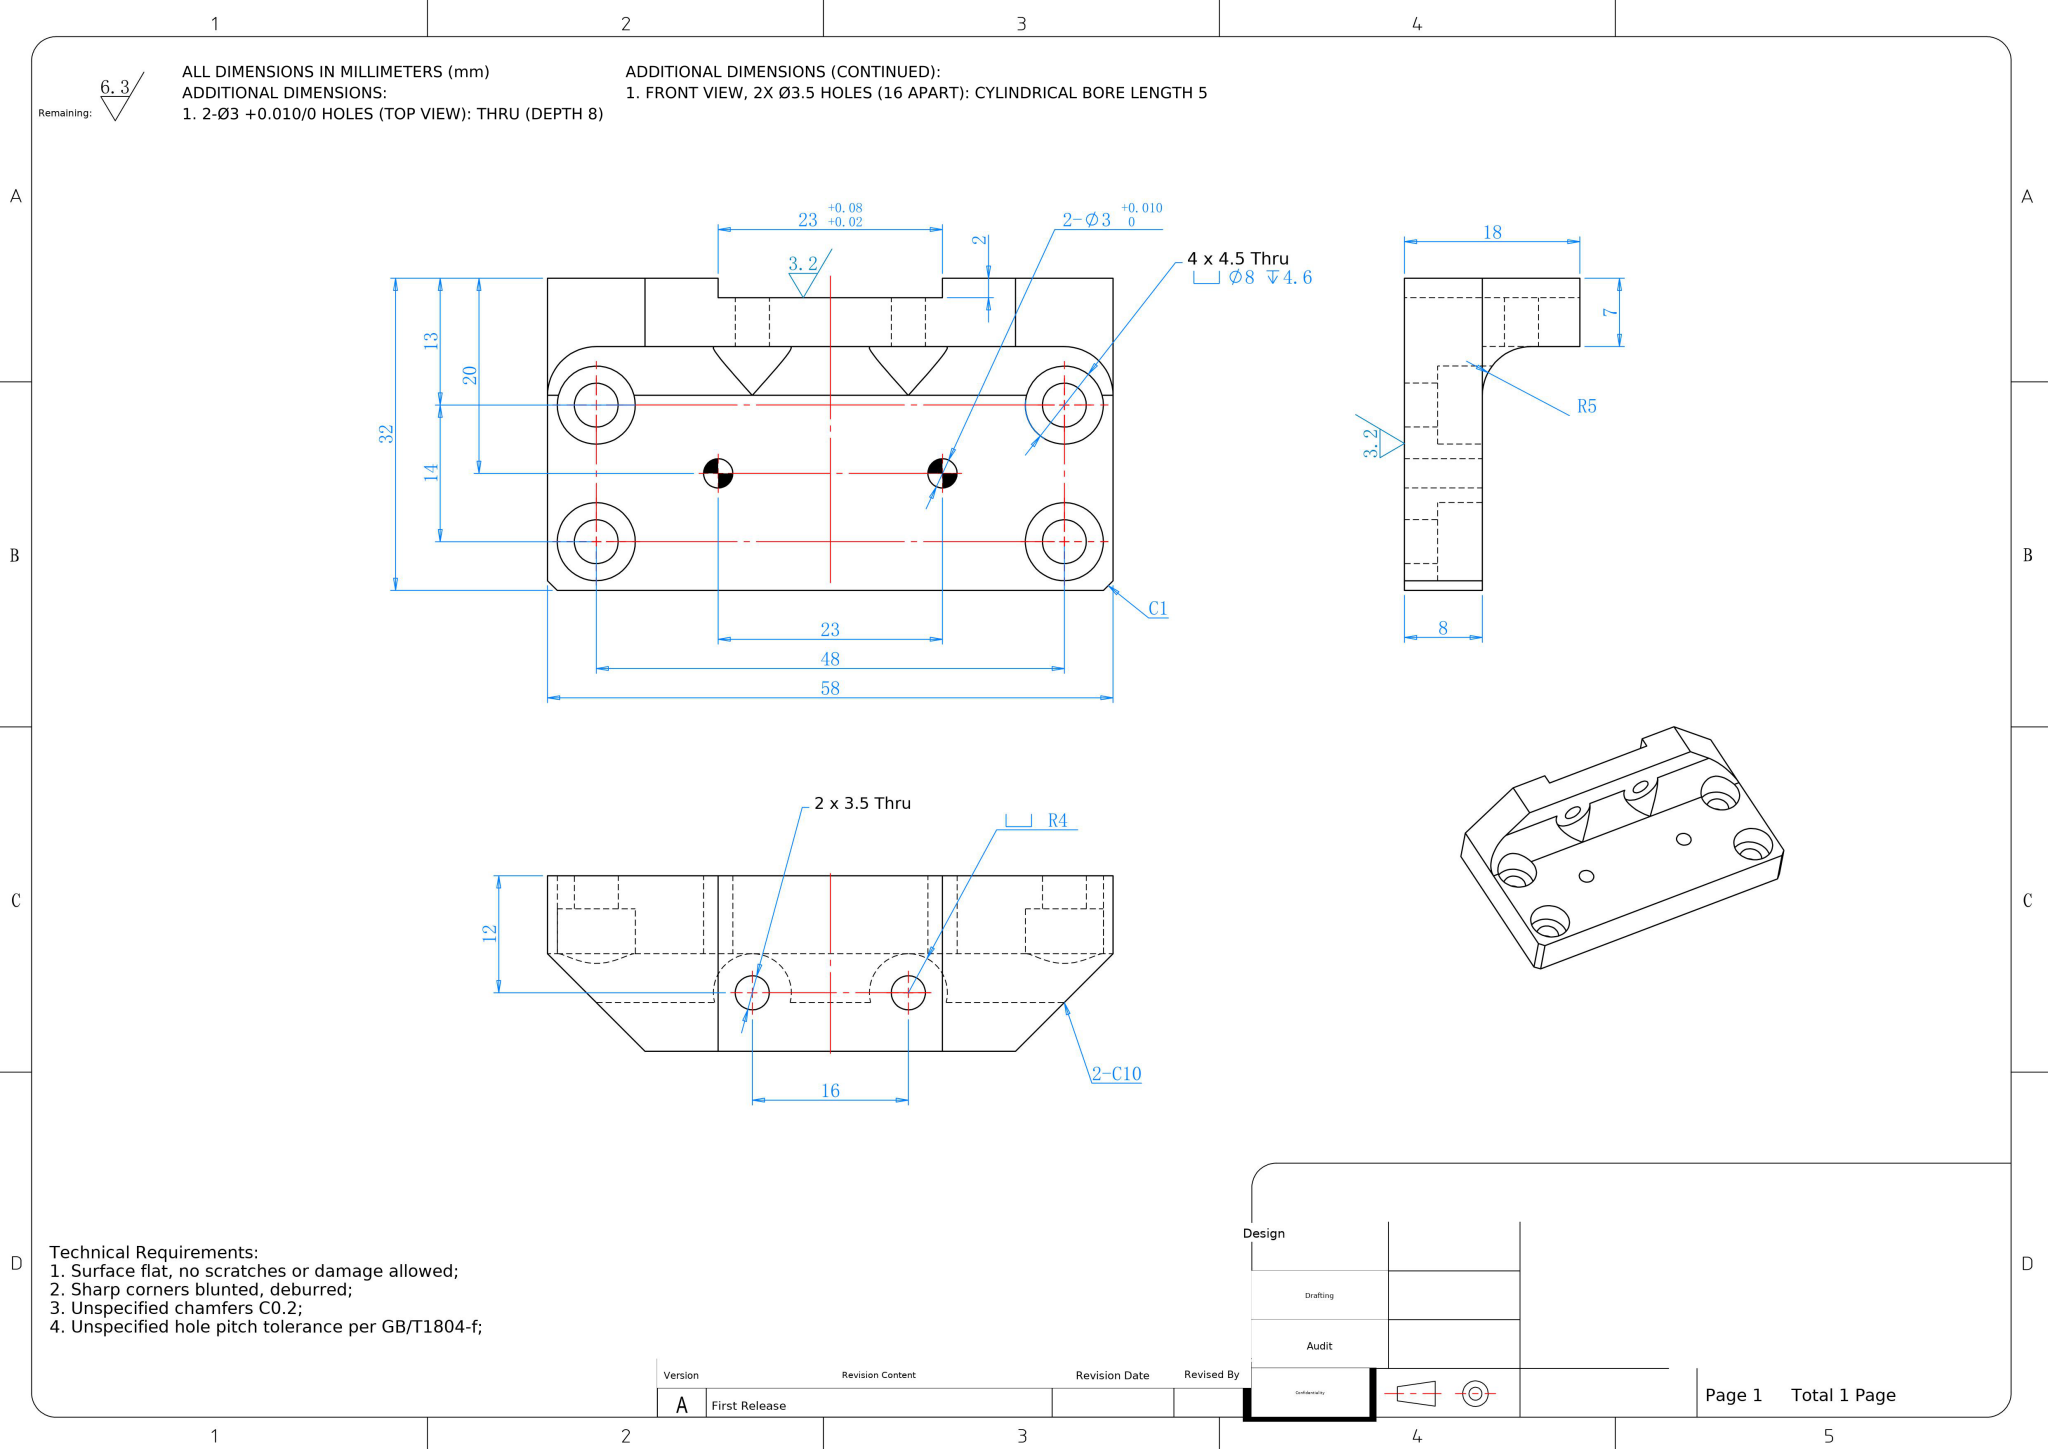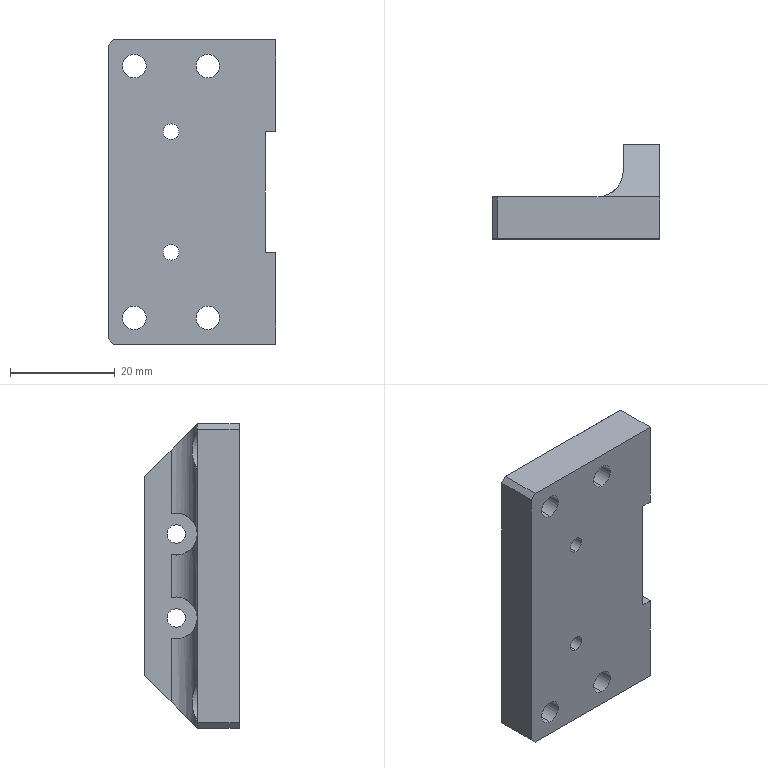Part | NX | mm | 1 solid | 49 faces | box 32 x 18 x 58 mm | volume 16261 mm3 | cylinder 29 | plane 20 | commonest cylinder face diameters 8 x10 4.5 x8 3 x4 3.5 x4 10 x3